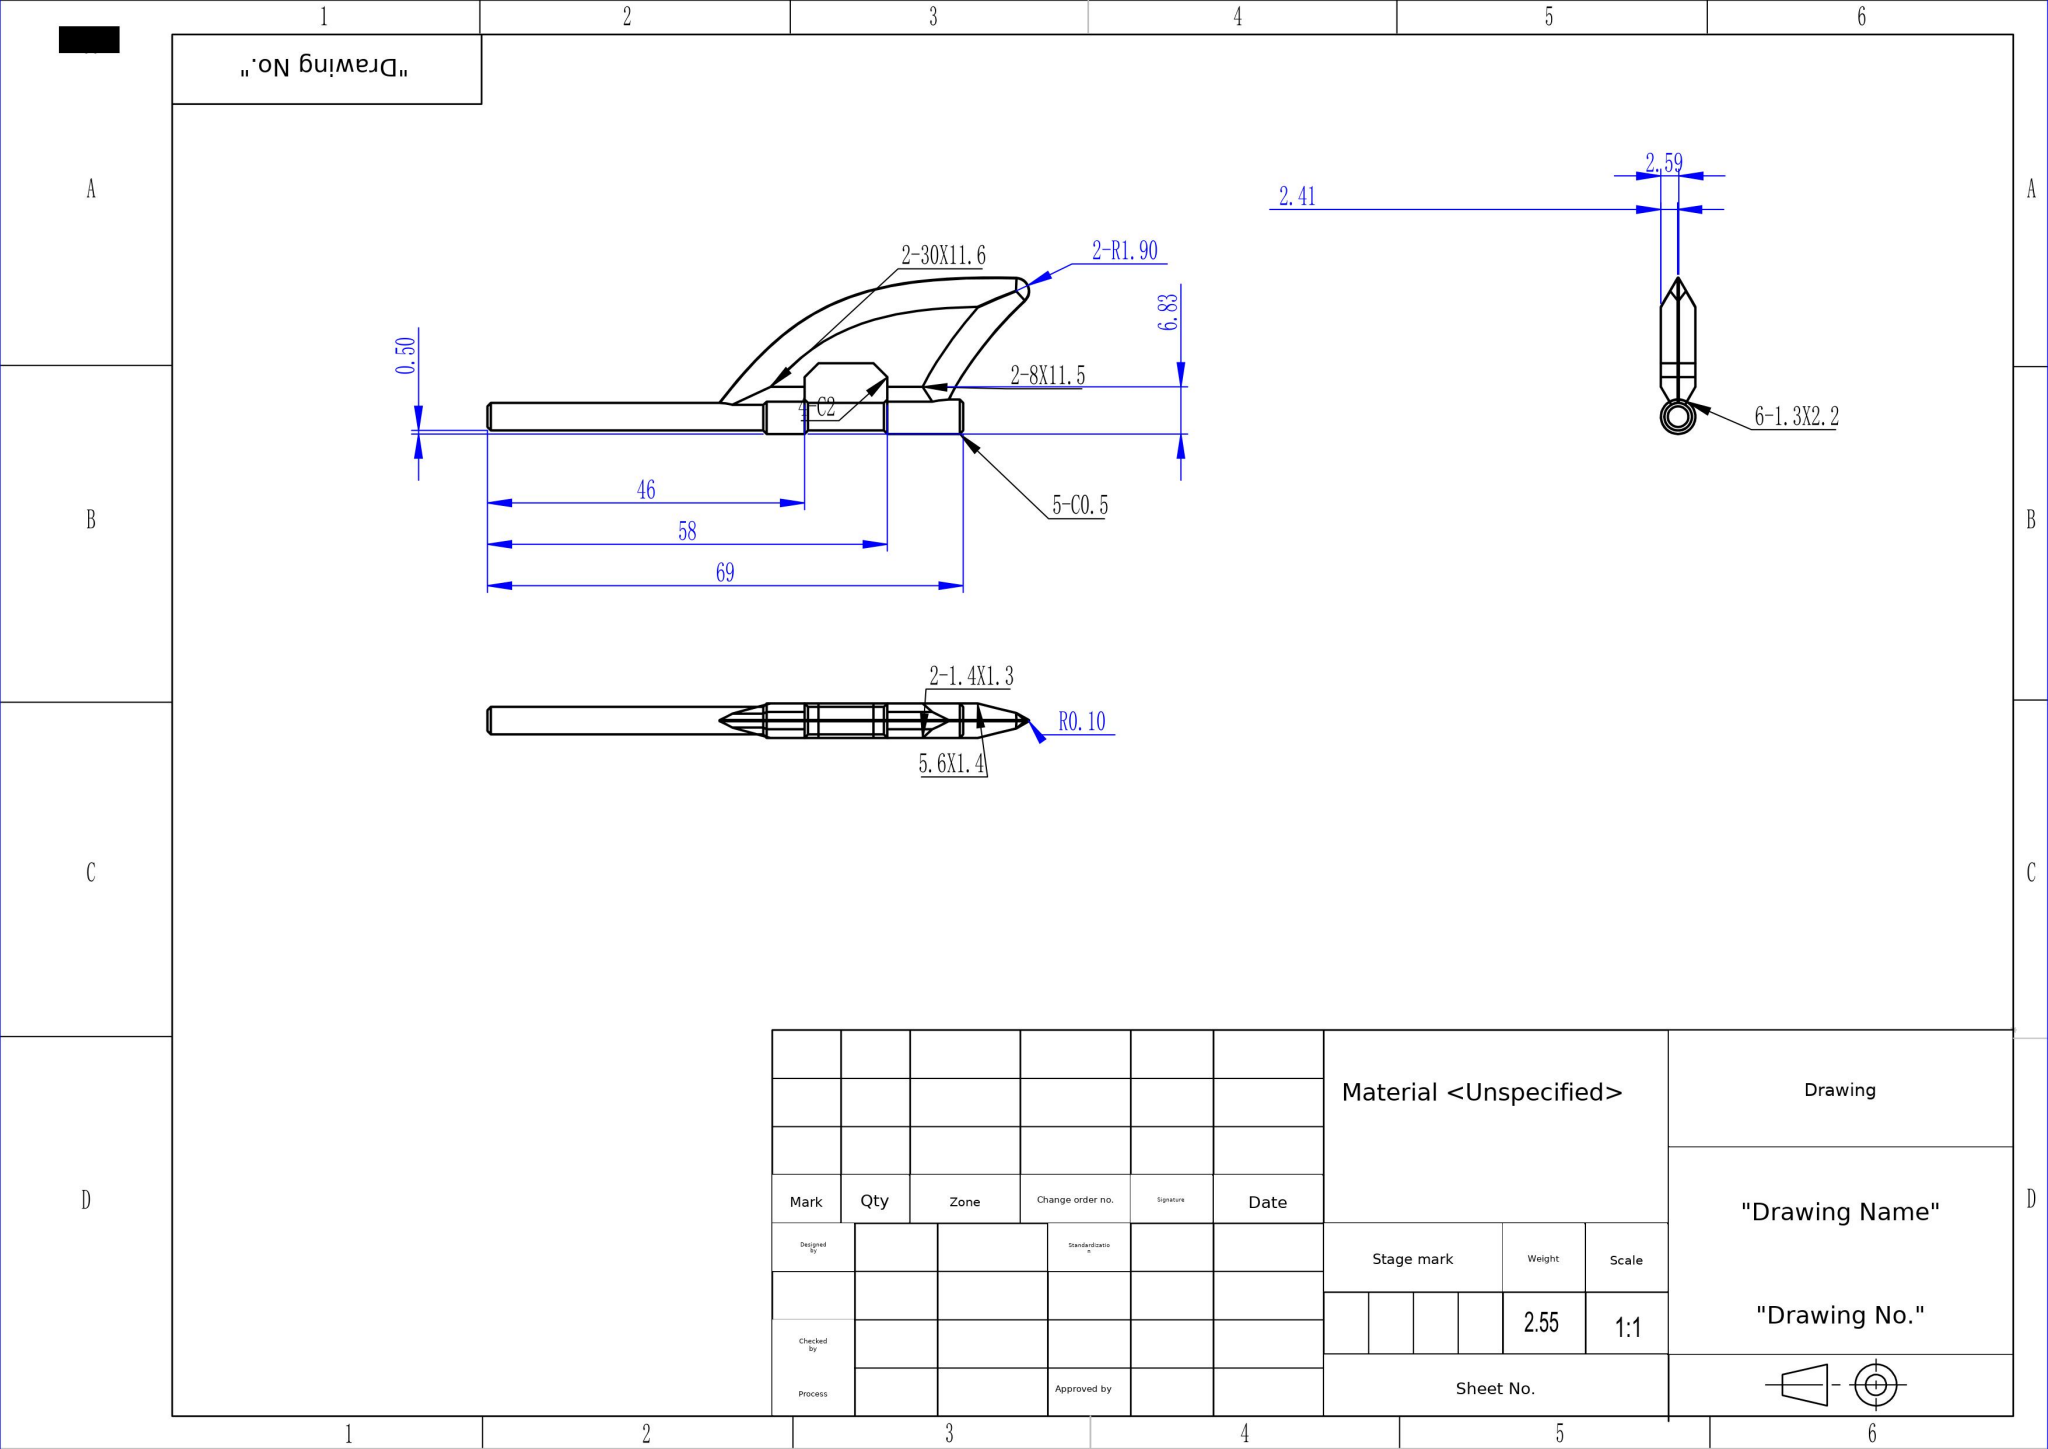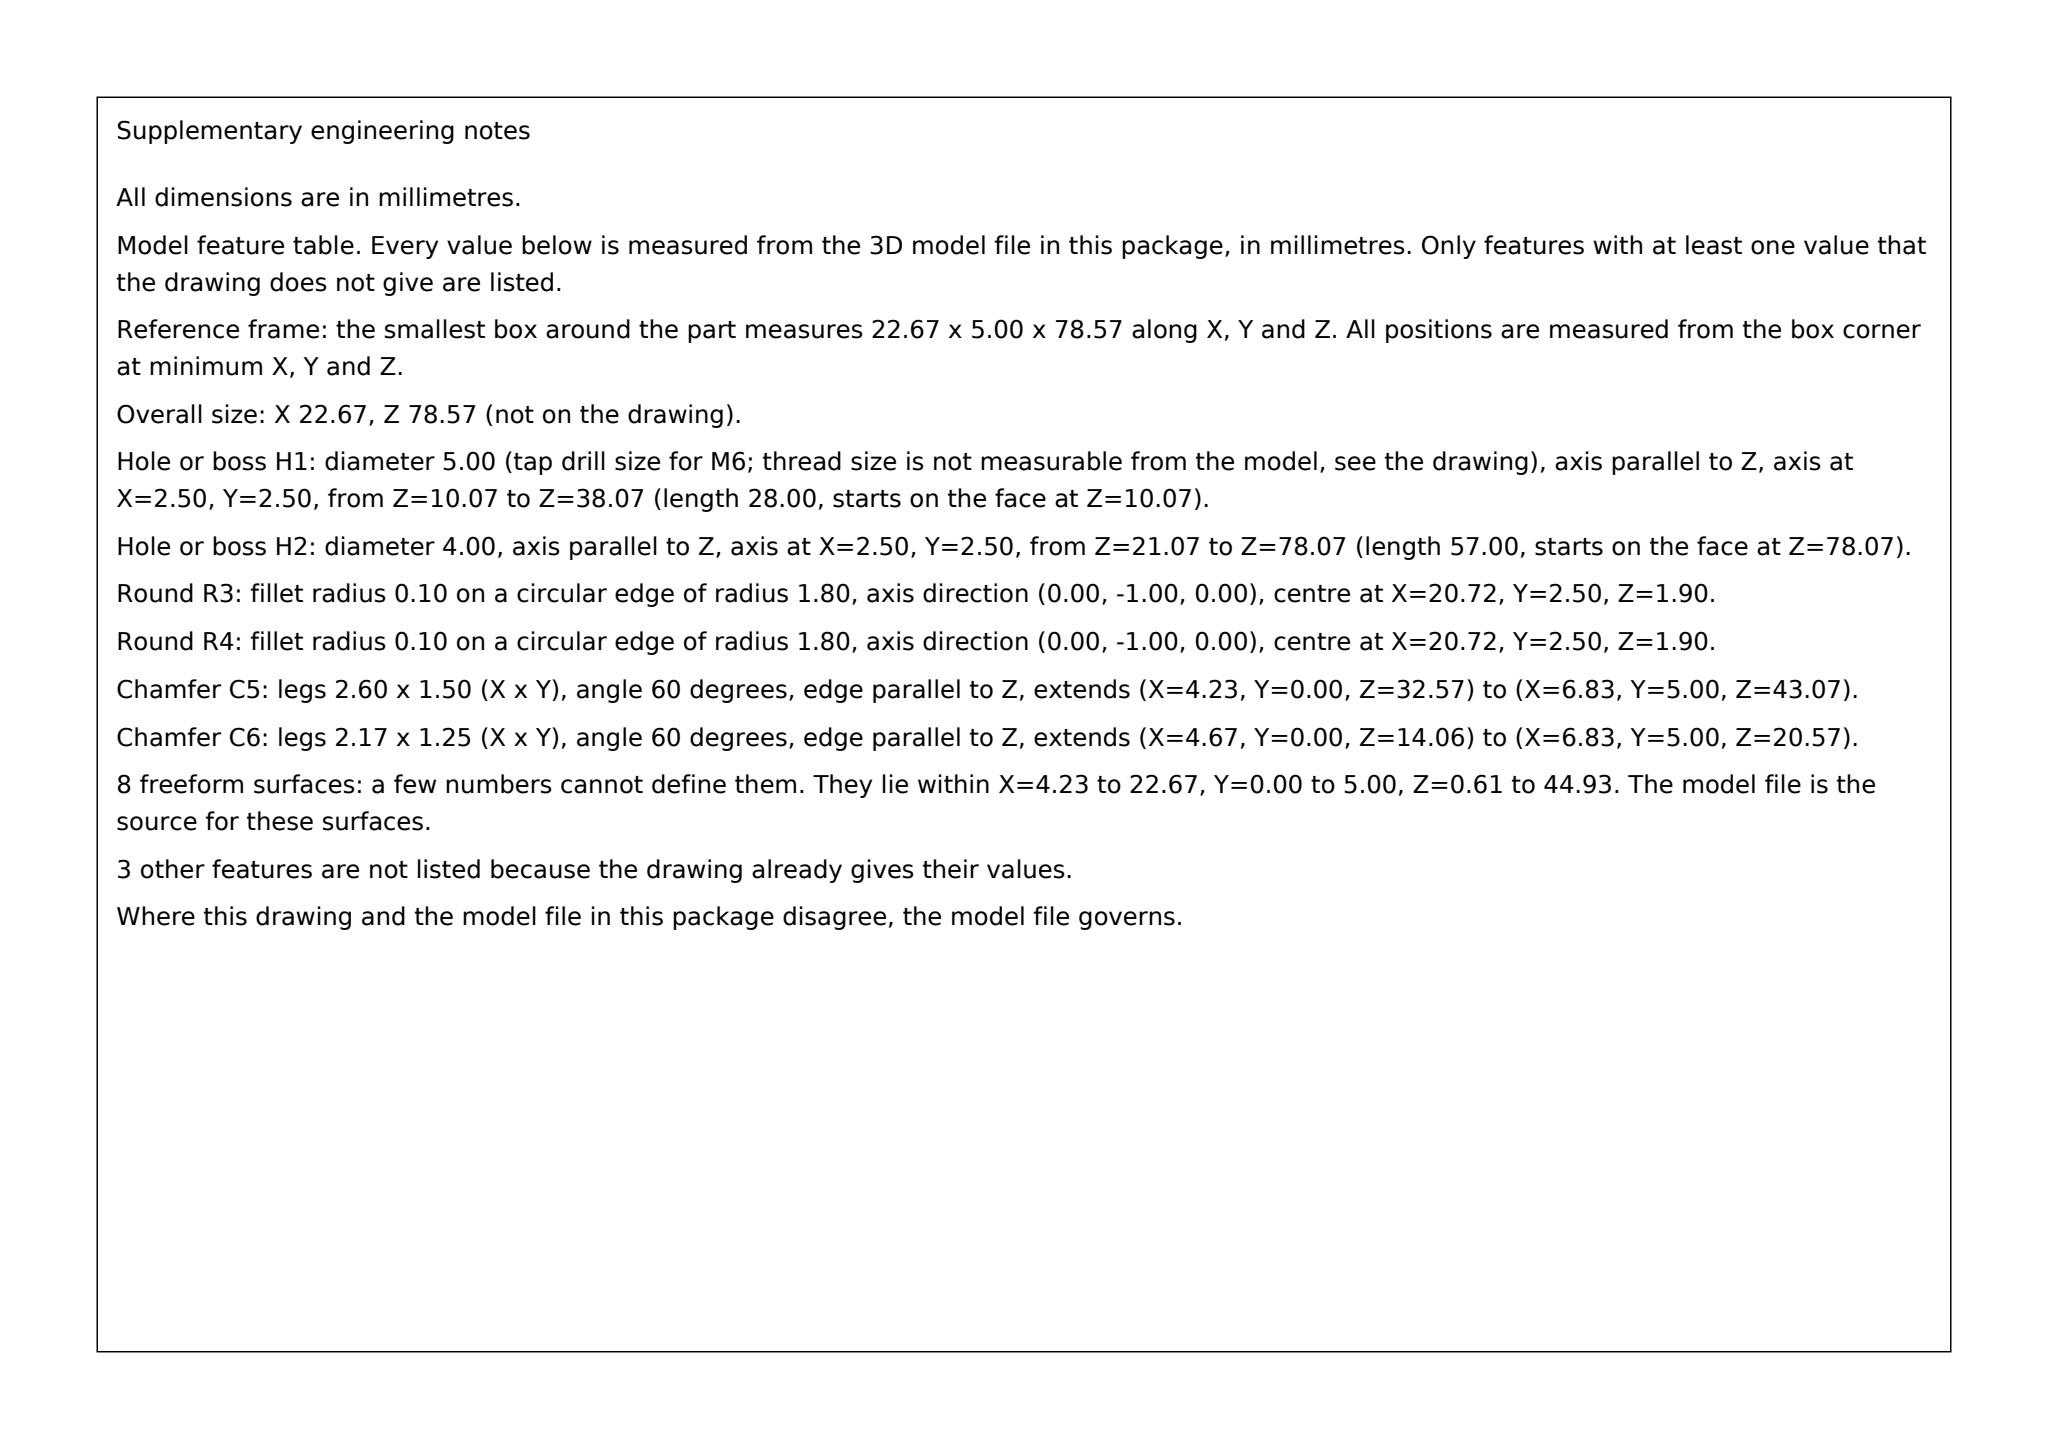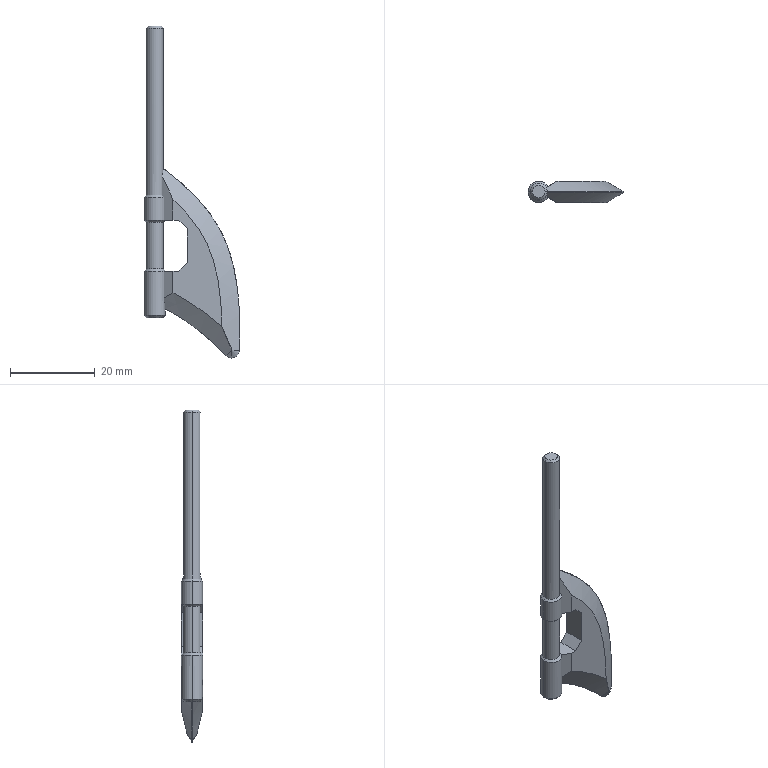Part | SolidWorks | mm | 1 solid | 45 faces | box 22.67 x 5 x 78.57 mm | volume 2551 mm3 | cone 14 | plane 13 | cylinder 8 | spline 8 | torus 2 | commonest cylinder face diameters 4 x4 5 x4